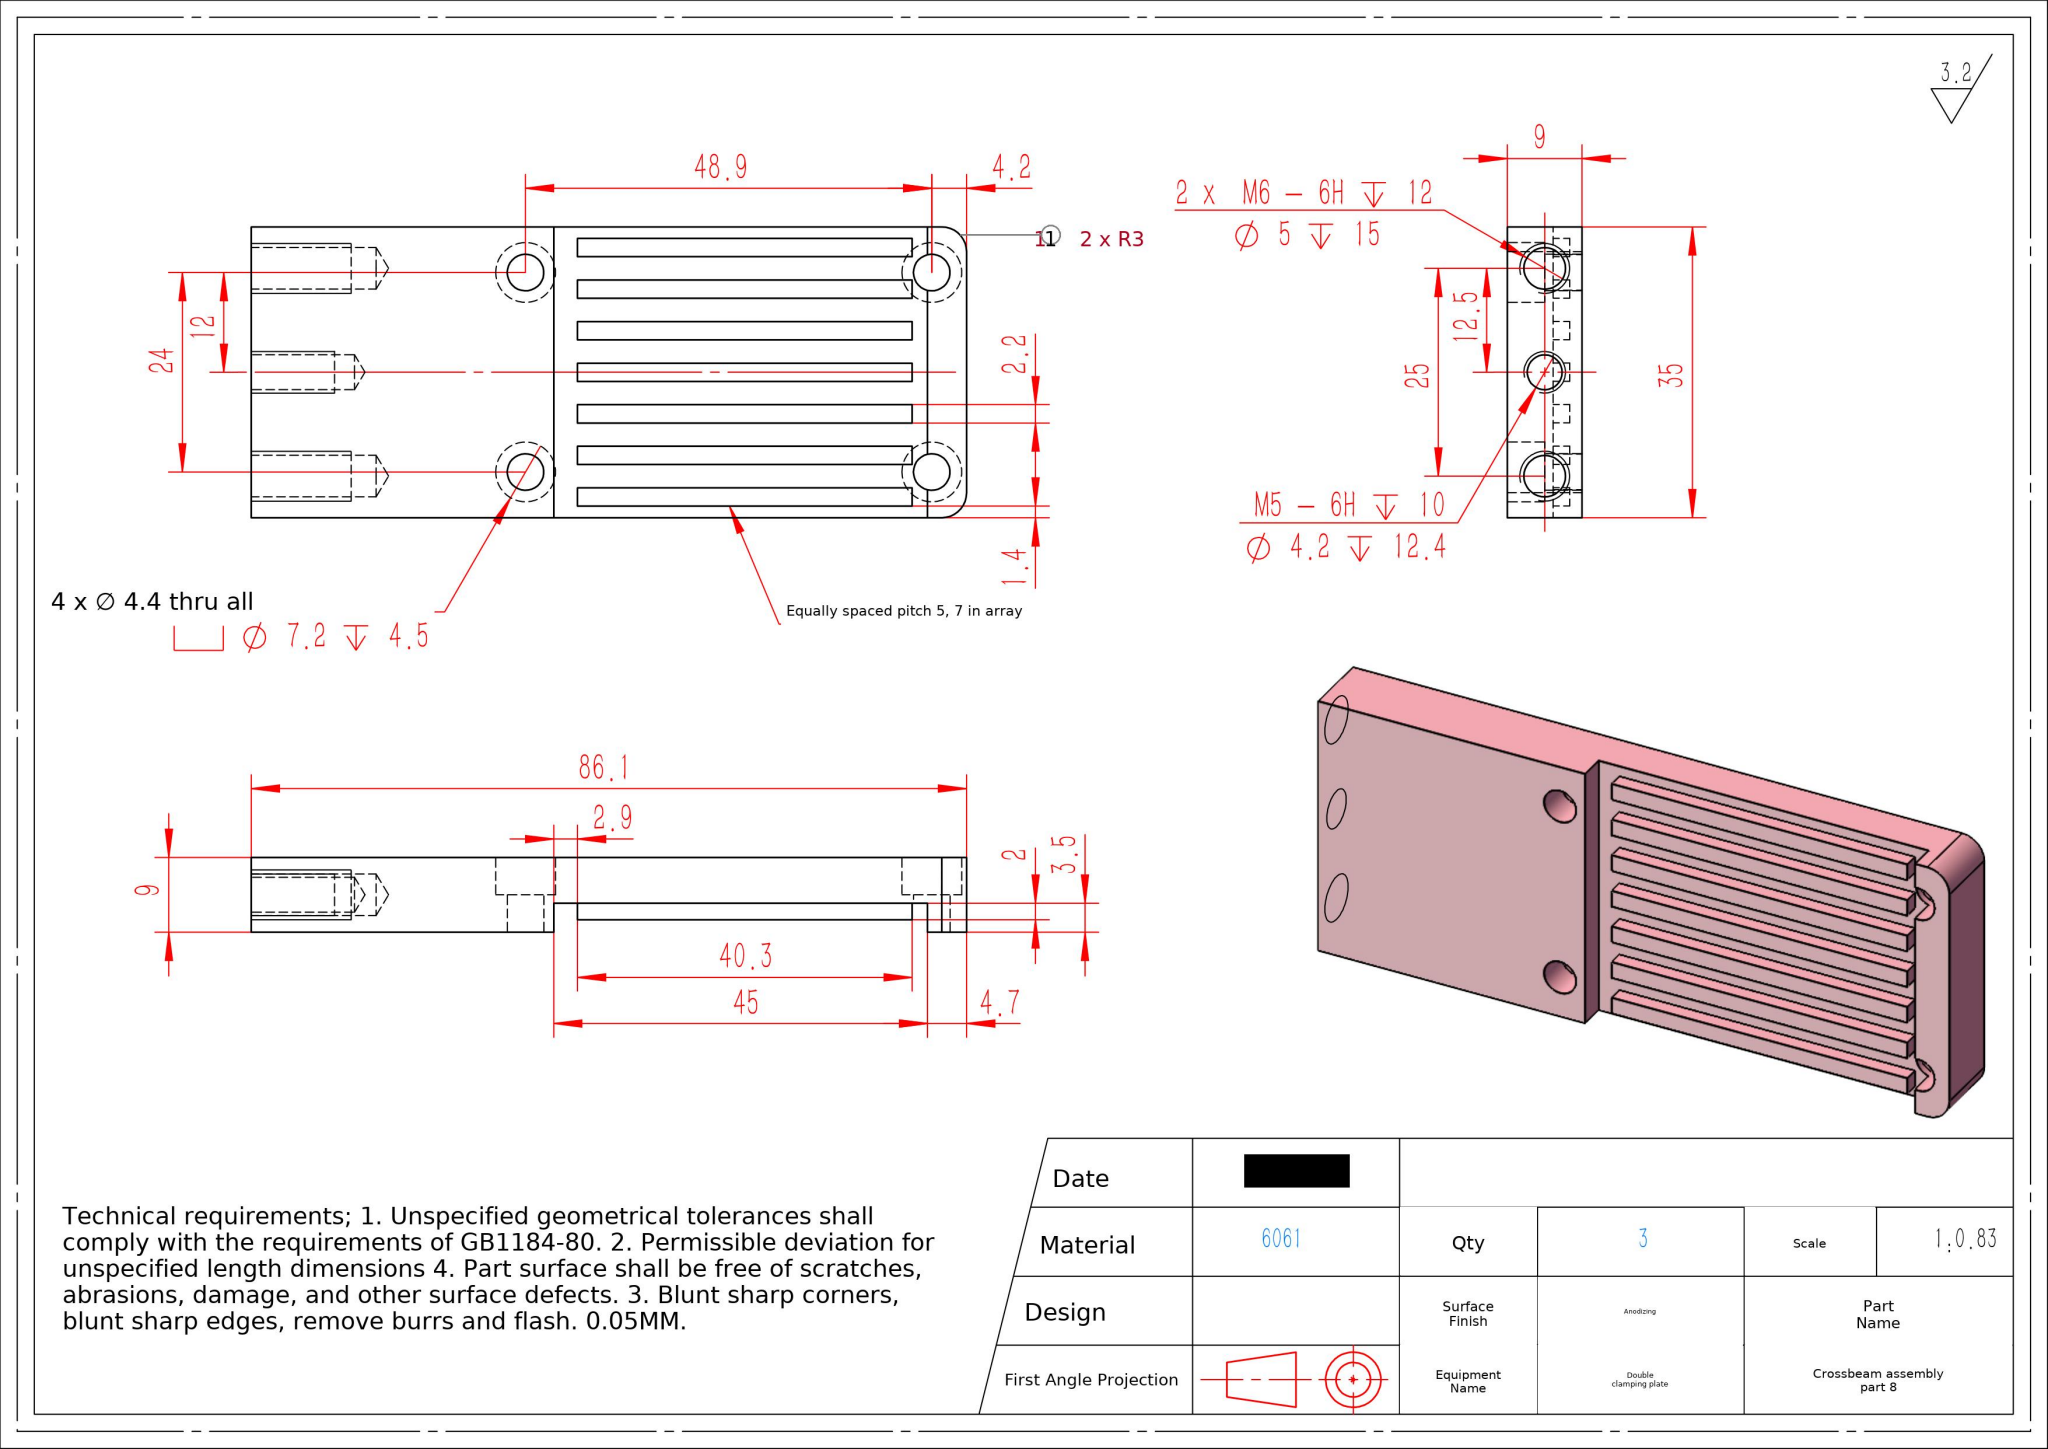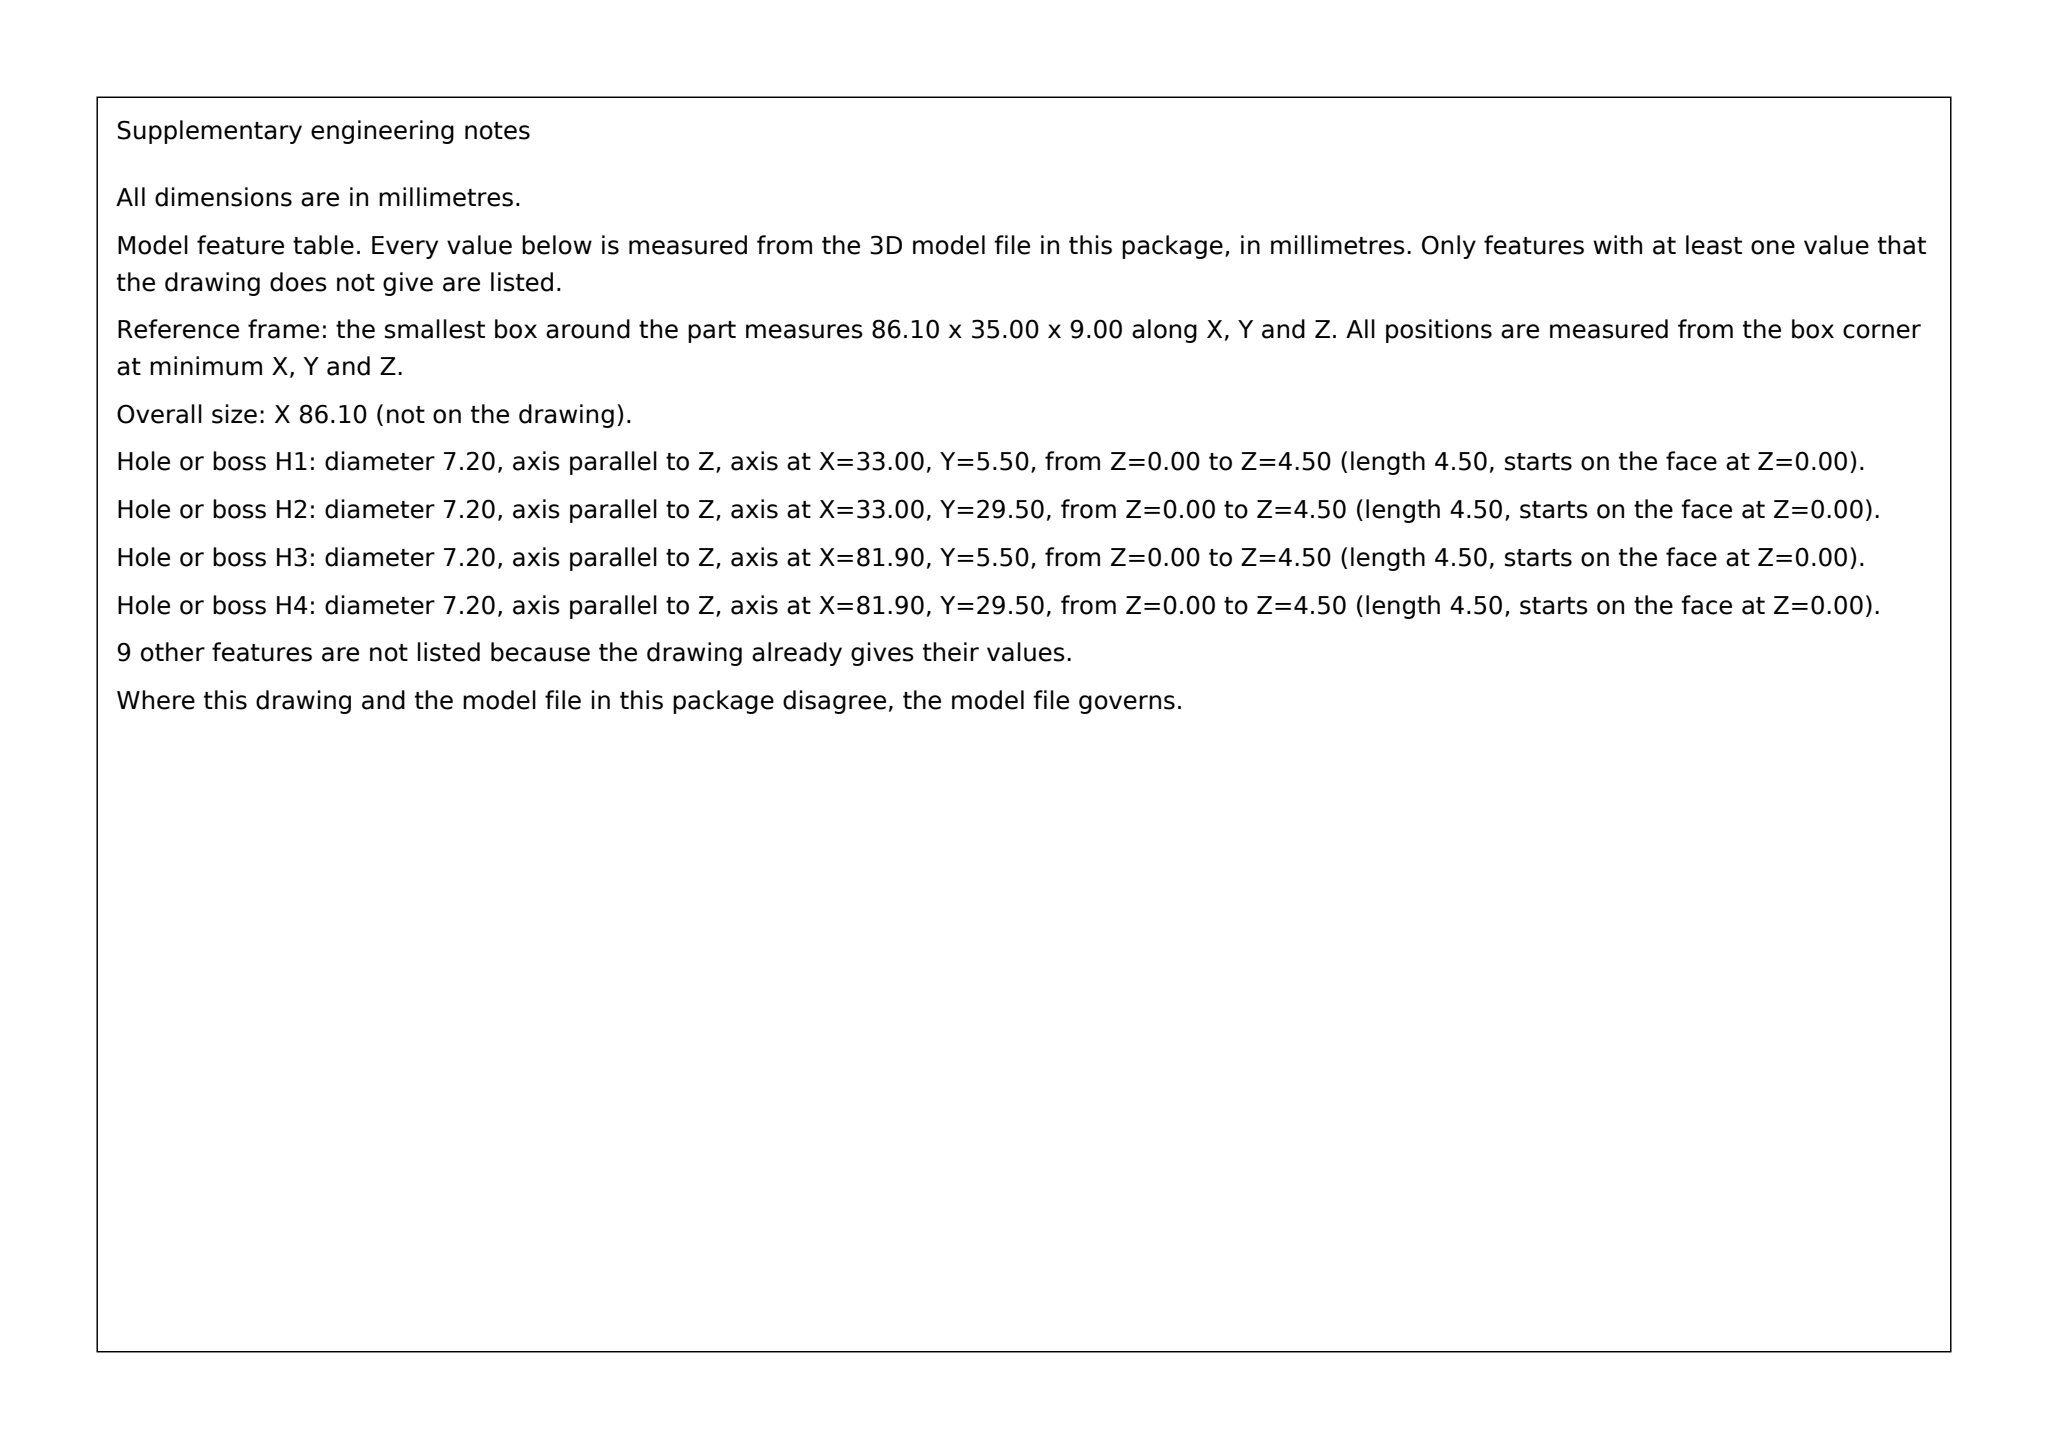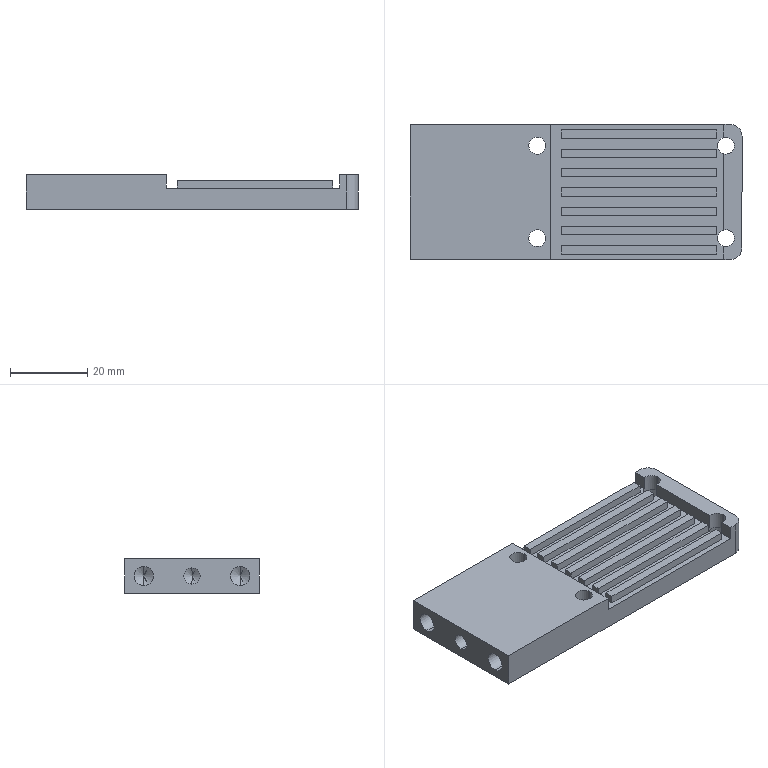Part | SolidWorks | mm | material 6061 | 1 solid | 81 faces | box 86.1 x 35 x 9 mm | volume 21061 mm3 | plane 51 | cylinder 24 | cone 6 | commonest cylinder face diameters 7.2 x8 4.4 x8 5 x4 4.2 x2 6 x2
build123d program:
from build123d import *

# Parameters (mm, degrees)
SKETCH1_W                                          = 86.1
SKETCH1_H                                          = 35
BOSS_EXTRUDE1_DEPTH                                = 9
SKETCH2_W                                          = 45
SKETCH2_H                                          = 3.5
CUT_EXTRUDE1_DEPTH                                 = 57.208
SKETCH3_W                                          = 40.3
SKETCH3_H                                          = 2.2
BOSS_EXTRUDE2_DEPTH                                = 2
M4_HEX_HEAD_MACHINE_SCREW_COUNTERBORE1_D           = 4.4
M4_HEX_HEAD_MACHINE_SCREW_COUNTERBORE1_CBORE_D     = 7.2
M4_HEX_HEAD_MACHINE_SCREW_COUNTERBORE1_CBORE_DEPTH = 4.5
M6_TAPPED_HOLE1_D                                  = 5
M6_TAPPED_HOLE1_DEPTH                              = 15
M6_TAPPED_HOLE1_TIP                                = 1.502
M5_TAPPED_HOLE1_D                                  = 4.2
M5_TAPPED_HOLE1_DEPTH                              = 12.4
M5_TAPPED_HOLE1_TIP                                = 1.262
FILLET1_R                                          = 3
LPATTERN1_COUNT                                    = 7
LPATTERN1_PITCH                                    = 5


with BuildPart() as part:
    # Sketch1 → Boss-Extrude1 (new body)
    with BuildSketch(Plane(origin=(0, 0, 0), x_dir=(-1, 0, 0), z_dir=(0, 0, -1))):
        Rectangle(SKETCH1_W, SKETCH1_H)
    extrude(amount=-BOSS_EXTRUDE1_DEPTH)

    # Sketch2 → Cut-Extrude1 (cut, through all)
    with BuildSketch(Plane(origin=(0, 17.5, 0), x_dir=(-1, 0, 0), z_dir=(0, 1, 0))):
        with Locations((-15.85, 7.25)):
            Rectangle(SKETCH2_W, SKETCH2_H)
    extrude(amount=-CUT_EXTRUDE1_DEPTH, mode=Mode.SUBTRACT)

    # Sketch3 → Boss-Extrude2 (add)
    with BuildSketch(Plane.XY.offset(5.5)):
        with Locations((16.35, -15)):
            Rectangle(SKETCH3_W, SKETCH3_H)
    boss_extrude2 = extrude(amount=BOSS_EXTRUDE2_DEPTH)

    # M4 Hex Head Machine Screw Counterbore1 (through all)
    with Locations(Plane(origin=(0, 0, 0), x_dir=(-1, 0, 0), z_dir=(0, 0, -1))):
        with Locations((-38.85, 12), (-38.85, -12), (10.05, 12), (10.05, -12)):
            CounterBoreHole(M4_HEX_HEAD_MACHINE_SCREW_COUNTERBORE1_D / 2, M4_HEX_HEAD_MACHINE_SCREW_COUNTERBORE1_CBORE_D / 2, M4_HEX_HEAD_MACHINE_SCREW_COUNTERBORE1_CBORE_DEPTH)

    # M6 Tapped Hole1
    with Locations(Plane.ZY.offset(43.05)):
        with Locations((4.5, 12.5), (4.5, -12.5)):
            Hole(M6_TAPPED_HOLE1_D / 2, depth=M6_TAPPED_HOLE1_DEPTH)
            with Locations((0, 0, -(M6_TAPPED_HOLE1_DEPTH + M6_TAPPED_HOLE1_TIP / 2))):  # 118° drill point
                Cone(0, M6_TAPPED_HOLE1_D / 2, M6_TAPPED_HOLE1_TIP, mode=Mode.SUBTRACT)

    # M5 Tapped Hole1
    with Locations(Plane.ZY.offset(43.05)):
        with Locations((4.5, 0)):
            Hole(M5_TAPPED_HOLE1_D / 2, depth=M5_TAPPED_HOLE1_DEPTH)
            with Locations((0, 0, -(M5_TAPPED_HOLE1_DEPTH + M5_TAPPED_HOLE1_TIP / 2))):  # 118° drill point
                Cone(0, M5_TAPPED_HOLE1_D / 2, M5_TAPPED_HOLE1_TIP, mode=Mode.SUBTRACT)

    # Fillet1
    fillet1_edges = [part.edges().sort_by_distance(p)[0] for p in [
        (43.05, 17.5, 4.5),
        (43.05, -17.5, 4.5),
    ]]
    fillet(fillet1_edges, radius=FILLET1_R)

    # LPattern1: Boss-Extrude2 ×7
    with Locations(*[(0, i * LPATTERN1_PITCH, 0) for i in range(1, LPATTERN1_COUNT)]):
        add(boss_extrude2)


solid = part.part